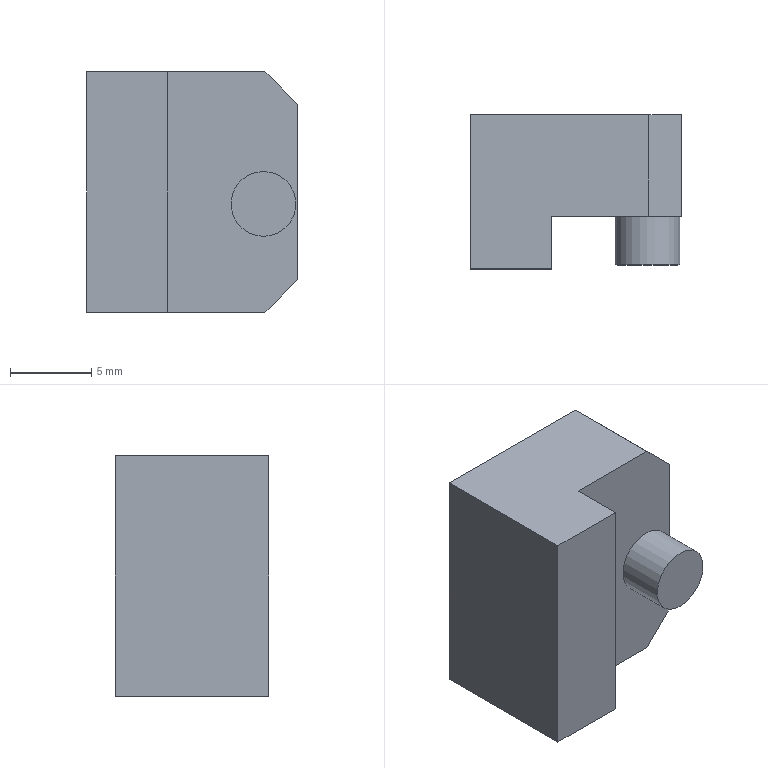Component | NX | SLIDER | 1 solid | 12 faces | box 13 x 9.5 x 14.83 mm | volume 1458 mm3 | plane 11 | cylinder 1 | commonest cylinder face diameters 4 x1
STEP:
#1=CARTESIAN_POINT('',(0.,0.,0.));
#2=DIRECTION('',(0.,0.,1.));
#3=DIRECTION('',(1.,0.,0.));
#4=AXIS2_PLACEMENT_3D('',#1,#2,#3);
#5=CARTESIAN_POINT('',(-316.,380.,341.346));
#6=VERTEX_POINT('',#5);
#7=CARTESIAN_POINT('',(-316.,380.,337.346));
#8=VERTEX_POINT('',#7);
#9=CARTESIAN_POINT('',(-316.,380.,339.346));
#10=DIRECTION('',(0.,-1.,0.));
#11=DIRECTION('',(0.,0.,1.));
#12=AXIS2_PLACEMENT_3D('',#9,#10,#11);
#13=CIRCLE('',#12,2.);
#14=CARTESIAN_POINT('',(-313.907,380.,347.493));
#15=DIRECTION('',(0.,1.,-0.));
#16=DIRECTION('',(0.,0.,1.));
#17=AXIS2_PLACEMENT_3D('',#14,#15,#16);
#18=PLANE('',#17);
#19=CARTESIAN_POINT('',(-6.147,-2.093));
#20=CARTESIAN_POINT('',(-6.147,-5.557));
#21=CARTESIAN_POINT('',(-9.147,-3.825));
#22=CARTESIAN_POINT('',(-12.147,-2.093));
#23=CARTESIAN_POINT('',(-9.147,-0.3606));
#24=CARTESIAN_POINT('',(-6.147,1.371));
#25=CARTESIAN_POINT('',(-6.147,-2.093));
#26=(BOUNDED_CURVE()B_SPLINE_CURVE(2,(#19,#20,#21,#22,#23,#24,#25),.UNSPECIFIED.,.T.,.F.)B_SPLINE_CURVE_WITH_KNOTS((1,2,2,2,2,1),(-2.094,0.,2.094,4.189,6.283,8.378),.UNSPECIFIED.)CURVE()GEOMETRIC_REPRESENTATION_ITEM()RATIONAL_B_SPLINE_CURVE((1.,0.5,1.,0.5,1.,0.5,1.))REPRESENTATION_ITEM(''));
#27=(GEOMETRIC_REPRESENTATION_CONTEXT(2)PARAMETRIC_REPRESENTATION_CONTEXT()REPRESENTATION_CONTEXT('',''));
#28=DEFINITIONAL_REPRESENTATION('',(#26),#27);
#29=PCURVE('',#18,#28);
#30=CARTESIAN_POINT('',(-316.,382.,339.346));
#31=DIRECTION('',(0.,-1.,-0.));
#32=DIRECTION('',(0.,0.,-1.));
#33=AXIS2_PLACEMENT_3D('',#30,#31,#32);
#34=CYLINDRICAL_SURFACE('',#33,2.);
#35=CARTESIAN_POINT('',(3.142,2.));
#36=DIRECTION('',(1.,0.));
#37=VECTOR('',#36,1.);
#38=LINE('',#35,#37);
#39=(GEOMETRIC_REPRESENTATION_CONTEXT(2)PARAMETRIC_REPRESENTATION_CONTEXT()REPRESENTATION_CONTEXT('',''));
#40=DEFINITIONAL_REPRESENTATION('',(#38),#39);
#41=PCURVE('',#34,#40);
#42=SURFACE_CURVE('',#13,(#29,#41),.PCURVE_S1.);
#43=EDGE_CURVE('',#6,#8,#42,.T.);
#44=ORIENTED_EDGE('',*,*,#43,.F.);
#45=CARTESIAN_POINT('',(-316.,380.,339.346));
#46=DIRECTION('',(0.,-1.,0.));
#47=DIRECTION('',(0.,0.,1.));
#48=AXIS2_PLACEMENT_3D('',#45,#46,#47);
#49=CIRCLE('',#48,2.);
#50=CARTESIAN_POINT('',(-6.147,-2.093));
#51=CARTESIAN_POINT('',(-6.147,-5.557));
#52=CARTESIAN_POINT('',(-9.147,-3.825));
#53=CARTESIAN_POINT('',(-12.147,-2.093));
#54=CARTESIAN_POINT('',(-9.147,-0.3606));
#55=CARTESIAN_POINT('',(-6.147,1.371));
#56=CARTESIAN_POINT('',(-6.147,-2.093));
#57=(BOUNDED_CURVE()B_SPLINE_CURVE(2,(#50,#51,#52,#53,#54,#55,#56),.UNSPECIFIED.,.T.,.F.)B_SPLINE_CURVE_WITH_KNOTS((1,2,2,2,2,1),(-2.094,0.,2.094,4.189,6.283,8.378),.UNSPECIFIED.)CURVE()GEOMETRIC_REPRESENTATION_ITEM()RATIONAL_B_SPLINE_CURVE((1.,0.5,1.,0.5,1.,0.5,1.))REPRESENTATION_ITEM(''));
#58=(GEOMETRIC_REPRESENTATION_CONTEXT(2)PARAMETRIC_REPRESENTATION_CONTEXT()REPRESENTATION_CONTEXT('',''));
#59=DEFINITIONAL_REPRESENTATION('',(#57),#58);
#60=PCURVE('',#18,#59);
#61=CARTESIAN_POINT('',(-3.142,2.));
#62=DIRECTION('',(1.,0.));
#63=VECTOR('',#62,1.);
#64=LINE('',#61,#63);
#65=(GEOMETRIC_REPRESENTATION_CONTEXT(2)PARAMETRIC_REPRESENTATION_CONTEXT()REPRESENTATION_CONTEXT('',''));
#66=DEFINITIONAL_REPRESENTATION('',(#64),#65);
#67=PCURVE('',#34,#66);
#68=SURFACE_CURVE('',#49,(#60,#67),.PCURVE_S1.);
#69=EDGE_CURVE('',#8,#6,#68,.T.);
#70=ORIENTED_EDGE('',*,*,#69,.F.);
#71=EDGE_LOOP('',(#44,#70));
#72=FACE_BOUND('',#71,.T.);
#73=CARTESIAN_POINT('',(-315.907,380.,332.665));
#74=VERTEX_POINT('',#73);
#75=CARTESIAN_POINT('',(-321.907,380.,332.665));
#76=VERTEX_POINT('',#75);
#77=CARTESIAN_POINT('',(-313.907,380.,332.665));
#78=DIRECTION('',(-1.,0.,0.));
#79=VECTOR('',#78,1.);
#80=LINE('',#77,#79);
#81=CARTESIAN_POINT('',(-14.828,0.));
#82=DIRECTION('',(0.,-1.));
#83=VECTOR('',#82,1.);
#84=LINE('',#81,#83);
#85=(GEOMETRIC_REPRESENTATION_CONTEXT(2)PARAMETRIC_REPRESENTATION_CONTEXT()REPRESENTATION_CONTEXT('',''));
#86=DEFINITIONAL_REPRESENTATION('',(#84),#85);
#87=PCURVE('',#18,#86);
#88=CARTESIAN_POINT('',(-313.907,380.,332.665));
#89=DIRECTION('',(0.,0.,1.));
#90=DIRECTION('',(-1.,0.,0.));
#91=AXIS2_PLACEMENT_3D('',#88,#89,#90);
#92=PLANE('',#91);
#93=CARTESIAN_POINT('',(0.,0.));
#94=DIRECTION('',(1.,0.));
#95=VECTOR('',#94,1.);
#96=LINE('',#93,#95);
#97=(GEOMETRIC_REPRESENTATION_CONTEXT(2)PARAMETRIC_REPRESENTATION_CONTEXT()REPRESENTATION_CONTEXT('',''));
#98=DEFINITIONAL_REPRESENTATION('',(#96),#97);
#99=PCURVE('',#92,#98);
#100=SURFACE_CURVE('',#80,(#87,#99),.PCURVE_S1.);
#101=EDGE_CURVE('',#74,#76,#100,.T.);
#102=ORIENTED_EDGE('',*,*,#101,.F.);
#103=CARTESIAN_POINT('',(-313.907,380.,334.665));
#104=VERTEX_POINT('',#103);
#105=CARTESIAN_POINT('',(-313.907,380.,334.665));
#106=DIRECTION('',(0.7071,0.,0.7071));
#107=VECTOR('',#106,1.);
#108=LINE('',#105,#107);
#109=CARTESIAN_POINT('',(-12.828,-0.));
#110=DIRECTION('',(0.7071,0.7071));
#111=VECTOR('',#110,1.);
#112=LINE('',#109,#111);
#113=(GEOMETRIC_REPRESENTATION_CONTEXT(2)PARAMETRIC_REPRESENTATION_CONTEXT()REPRESENTATION_CONTEXT('',''));
#114=DEFINITIONAL_REPRESENTATION('',(#112),#113);
#115=PCURVE('',#18,#114);
#116=CARTESIAN_POINT('',(-313.907,0.,334.665));
#117=DIRECTION('',(0.7071,0.,-0.7071));
#118=DIRECTION('',(0.,-1.,0.));
#119=AXIS2_PLACEMENT_3D('',#116,#117,#118);
#120=PLANE('',#119);
#121=CARTESIAN_POINT('',(-380.,0.));
#122=DIRECTION('',(-0.,-1.));
#123=VECTOR('',#122,1.);
#124=LINE('',#121,#123);
#125=(GEOMETRIC_REPRESENTATION_CONTEXT(2)PARAMETRIC_REPRESENTATION_CONTEXT()REPRESENTATION_CONTEXT('',''));
#126=DEFINITIONAL_REPRESENTATION('',(#124),#125);
#127=PCURVE('',#120,#126);
#128=SURFACE_CURVE('',#108,(#115,#127),.PCURVE_S1.);
#129=EDGE_CURVE('',#74,#104,#128,.T.);
#130=ORIENTED_EDGE('',*,*,#129,.T.);
#131=CARTESIAN_POINT('',(-313.907,380.,345.493));
#132=VERTEX_POINT('',#131);
#133=CARTESIAN_POINT('',(-313.907,380.,347.493));
#134=DIRECTION('',(0.,-0.,-1.));
#135=VECTOR('',#134,1.);
#136=LINE('',#133,#135);
#137=CARTESIAN_POINT('',(0.,0.));
#138=DIRECTION('',(-1.,0.));
#139=VECTOR('',#138,1.);
#140=LINE('',#137,#139);
#141=(GEOMETRIC_REPRESENTATION_CONTEXT(2)PARAMETRIC_REPRESENTATION_CONTEXT()REPRESENTATION_CONTEXT('',''));
#142=DEFINITIONAL_REPRESENTATION('',(#140),#141);
#143=PCURVE('',#18,#142);
#144=CARTESIAN_POINT('',(-313.907,0.,678.691));
#145=DIRECTION('',(1.,0.,0.));
#146=DIRECTION('',(0.,0.,1.));
#147=AXIS2_PLACEMENT_3D('',#144,#145,#146);
#148=PLANE('',#147);
#149=CARTESIAN_POINT('',(-331.198,-380.));
#150=DIRECTION('',(-1.,0.));
#151=VECTOR('',#150,1.);
#152=LINE('',#149,#151);
#153=(GEOMETRIC_REPRESENTATION_CONTEXT(2)PARAMETRIC_REPRESENTATION_CONTEXT()REPRESENTATION_CONTEXT('',''));
#154=DEFINITIONAL_REPRESENTATION('',(#152),#153);
#155=PCURVE('',#148,#154);
#156=SURFACE_CURVE('',#136,(#143,#155),.PCURVE_S1.);
#157=EDGE_CURVE('',#132,#104,#156,.T.);
#158=ORIENTED_EDGE('',*,*,#157,.F.);
#159=CARTESIAN_POINT('',(-315.907,380.,347.493));
#160=VERTEX_POINT('',#159);
#161=CARTESIAN_POINT('',(-313.907,380.,345.493));
#162=DIRECTION('',(-0.7071,0.,0.7071));
#163=VECTOR('',#162,1.);
#164=LINE('',#161,#163);
#165=CARTESIAN_POINT('',(-2.,0.));
#166=DIRECTION('',(0.7071,-0.7071));
#167=VECTOR('',#166,1.);
#168=LINE('',#165,#167);
#169=(GEOMETRIC_REPRESENTATION_CONTEXT(2)PARAMETRIC_REPRESENTATION_CONTEXT()REPRESENTATION_CONTEXT('',''));
#170=DEFINITIONAL_REPRESENTATION('',(#168),#169);
#171=PCURVE('',#18,#170);
#172=CARTESIAN_POINT('',(-313.907,0.,345.493));
#173=DIRECTION('',(0.7071,0.,0.7071));
#174=DIRECTION('',(0.,1.,0.));
#175=AXIS2_PLACEMENT_3D('',#172,#173,#174);
#176=PLANE('',#175);
#177=CARTESIAN_POINT('',(380.,-0.));
#178=DIRECTION('',(0.,1.));
#179=VECTOR('',#178,1.);
#180=LINE('',#177,#179);
#181=(GEOMETRIC_REPRESENTATION_CONTEXT(2)PARAMETRIC_REPRESENTATION_CONTEXT()REPRESENTATION_CONTEXT('',''));
#182=DEFINITIONAL_REPRESENTATION('',(#180),#181);
#183=PCURVE('',#176,#182);
#184=SURFACE_CURVE('',#164,(#171,#183),.PCURVE_S1.);
#185=EDGE_CURVE('',#132,#160,#184,.T.);
#186=ORIENTED_EDGE('',*,*,#185,.T.);
#187=CARTESIAN_POINT('',(-321.907,380.,347.493));
#188=VERTEX_POINT('',#187);
#189=CARTESIAN_POINT('',(-313.907,380.,347.493));
#190=DIRECTION('',(-1.,0.,0.));
#191=VECTOR('',#190,1.);
#192=LINE('',#189,#191);
#193=CARTESIAN_POINT('',(0.,0.));
#194=DIRECTION('',(0.,-1.));
#195=VECTOR('',#194,1.);
#196=LINE('',#193,#195);
#197=(GEOMETRIC_REPRESENTATION_CONTEXT(2)PARAMETRIC_REPRESENTATION_CONTEXT()REPRESENTATION_CONTEXT('',''));
#198=DEFINITIONAL_REPRESENTATION('',(#196),#197);
#199=PCURVE('',#18,#198);
#200=CARTESIAN_POINT('',(-313.907,386.248,347.493));
#201=DIRECTION('',(0.,0.,-1.));
#202=DIRECTION('',(1.,0.,0.));
#203=AXIS2_PLACEMENT_3D('',#200,#201,#202);
#204=PLANE('',#203);
#205=CARTESIAN_POINT('',(0.,6.248));
#206=DIRECTION('',(-1.,0.));
#207=VECTOR('',#206,1.);
#208=LINE('',#205,#207);
#209=(GEOMETRIC_REPRESENTATION_CONTEXT(2)PARAMETRIC_REPRESENTATION_CONTEXT()REPRESENTATION_CONTEXT('',''));
#210=DEFINITIONAL_REPRESENTATION('',(#208),#209);
#211=PCURVE('',#204,#210);
#212=SURFACE_CURVE('',#192,(#199,#211),.PCURVE_S1.);
#213=EDGE_CURVE('',#160,#188,#212,.T.);
#214=ORIENTED_EDGE('',*,*,#213,.T.);
#215=CARTESIAN_POINT('',(-321.907,380.,332.665));
#216=DIRECTION('',(0.,0.,1.));
#217=VECTOR('',#216,1.);
#218=LINE('',#215,#217);
#219=CARTESIAN_POINT('',(-14.828,-8.));
#220=DIRECTION('',(1.,0.));
#221=VECTOR('',#220,1.);
#222=LINE('',#219,#221);
#223=(GEOMETRIC_REPRESENTATION_CONTEXT(2)PARAMETRIC_REPRESENTATION_CONTEXT()REPRESENTATION_CONTEXT('',''));
#224=DEFINITIONAL_REPRESENTATION('',(#222),#223);
#225=PCURVE('',#18,#224);
#226=CARTESIAN_POINT('',(-321.907,0.,678.691));
#227=DIRECTION('',(1.,0.,0.));
#228=DIRECTION('',(0.,0.,1.));
#229=AXIS2_PLACEMENT_3D('',#226,#227,#228);
#230=PLANE('',#229);
#231=CARTESIAN_POINT('',(-346.026,-380.));
#232=DIRECTION('',(1.,-0.));
#233=VECTOR('',#232,1.);
#234=LINE('',#231,#233);
#235=(GEOMETRIC_REPRESENTATION_CONTEXT(2)PARAMETRIC_REPRESENTATION_CONTEXT()REPRESENTATION_CONTEXT('',''));
#236=DEFINITIONAL_REPRESENTATION('',(#234),#235);
#237=PCURVE('',#230,#236);
#238=SURFACE_CURVE('',#218,(#225,#237),.PCURVE_S1.);
#239=EDGE_CURVE('',#76,#188,#238,.T.);
#240=ORIENTED_EDGE('',*,*,#239,.F.);
#241=EDGE_LOOP('',(#102,#130,#158,#186,#214,#240));
#242=FACE_BOUND('',#241,.T.);
#243=ADVANCED_FACE('',(#72,#242),#18,.F.);
#244=CARTESIAN_POINT('',(-313.907,386.248,334.665));
#245=VERTEX_POINT('',#244);
#246=CARTESIAN_POINT('',(-313.907,386.248,345.493));
#247=VERTEX_POINT('',#246);
#248=CARTESIAN_POINT('',(-313.907,386.248,332.665));
#249=DIRECTION('',(0.,0.,1.));
#250=VECTOR('',#249,1.);
#251=LINE('',#248,#250);
#252=CARTESIAN_POINT('',(-313.907,386.248,332.665));
#253=DIRECTION('',(0.,-1.,0.));
#254=DIRECTION('',(0.,0.,-1.));
#255=AXIS2_PLACEMENT_3D('',#252,#253,#254);
#256=PLANE('',#255);
#257=CARTESIAN_POINT('',(0.,0.));
#258=DIRECTION('',(-1.,0.));
#259=VECTOR('',#258,1.);
#260=LINE('',#257,#259);
#261=(GEOMETRIC_REPRESENTATION_CONTEXT(2)PARAMETRIC_REPRESENTATION_CONTEXT()REPRESENTATION_CONTEXT('',''));
#262=DEFINITIONAL_REPRESENTATION('',(#260),#261);
#263=PCURVE('',#256,#262);
#264=CARTESIAN_POINT('',(-346.026,-386.248));
#265=DIRECTION('',(1.,0.));
#266=VECTOR('',#265,1.);
#267=LINE('',#264,#266);
#268=(GEOMETRIC_REPRESENTATION_CONTEXT(2)PARAMETRIC_REPRESENTATION_CONTEXT()REPRESENTATION_CONTEXT('',''));
#269=DEFINITIONAL_REPRESENTATION('',(#267),#268);
#270=PCURVE('',#148,#269);
#271=SURFACE_CURVE('',#251,(#263,#270),.PCURVE_S1.);
#272=EDGE_CURVE('',#245,#247,#271,.T.);
#273=ORIENTED_EDGE('',*,*,#272,.F.);
#274=CARTESIAN_POINT('',(-315.907,386.248,332.665));
#275=VERTEX_POINT('',#274);
#276=CARTESIAN_POINT('',(-313.907,386.248,334.665));
#277=DIRECTION('',(-0.7071,0.,-0.7071));
#278=VECTOR('',#277,1.);
#279=LINE('',#276,#278);
#280=CARTESIAN_POINT('',(-2.,0.));
#281=DIRECTION('',(0.7071,-0.7071));
#282=VECTOR('',#281,1.);
#283=LINE('',#280,#282);
#284=(GEOMETRIC_REPRESENTATION_CONTEXT(2)PARAMETRIC_REPRESENTATION_CONTEXT()REPRESENTATION_CONTEXT('',''));
#285=DEFINITIONAL_REPRESENTATION('',(#283),#284);
#286=PCURVE('',#256,#285);
#287=CARTESIAN_POINT('',(-386.248,0.));
#288=DIRECTION('',(0.,1.));
#289=VECTOR('',#288,1.);
#290=LINE('',#287,#289);
#291=(GEOMETRIC_REPRESENTATION_CONTEXT(2)PARAMETRIC_REPRESENTATION_CONTEXT()REPRESENTATION_CONTEXT('',''));
#292=DEFINITIONAL_REPRESENTATION('',(#290),#291);
#293=PCURVE('',#120,#292);
#294=SURFACE_CURVE('',#279,(#286,#293),.PCURVE_S1.);
#295=EDGE_CURVE('',#245,#275,#294,.T.);
#296=ORIENTED_EDGE('',*,*,#295,.T.);
#297=CARTESIAN_POINT('',(-326.907,386.248,332.665));
#298=VERTEX_POINT('',#297);
#299=CARTESIAN_POINT('',(-313.907,386.248,332.665));
#300=DIRECTION('',(-1.,0.,0.));
#301=VECTOR('',#300,1.);
#302=LINE('',#299,#301);
#303=CARTESIAN_POINT('',(0.,0.));
#304=DIRECTION('',(0.,-1.));
#305=VECTOR('',#304,1.);
#306=LINE('',#303,#305);
#307=(GEOMETRIC_REPRESENTATION_CONTEXT(2)PARAMETRIC_REPRESENTATION_CONTEXT()REPRESENTATION_CONTEXT('',''));
#308=DEFINITIONAL_REPRESENTATION('',(#306),#307);
#309=PCURVE('',#256,#308);
#310=CARTESIAN_POINT('',(0.,-6.248));
#311=DIRECTION('',(1.,0.));
#312=VECTOR('',#311,1.);
#313=LINE('',#310,#312);
#314=(GEOMETRIC_REPRESENTATION_CONTEXT(2)PARAMETRIC_REPRESENTATION_CONTEXT()REPRESENTATION_CONTEXT('',''));
#315=DEFINITIONAL_REPRESENTATION('',(#313),#314);
#316=PCURVE('',#92,#315);
#317=SURFACE_CURVE('',#302,(#309,#316),.PCURVE_S1.);
#318=EDGE_CURVE('',#275,#298,#317,.T.);
#319=ORIENTED_EDGE('',*,*,#318,.T.);
#320=CARTESIAN_POINT('',(-326.907,386.248,347.493));
#321=VERTEX_POINT('',#320);
#322=CARTESIAN_POINT('',(-326.907,386.248,332.665));
#323=DIRECTION('',(0.,0.,1.));
#324=VECTOR('',#323,1.);
#325=LINE('',#322,#324);
#326=CARTESIAN_POINT('',(0.,-13.));
#327=DIRECTION('',(-1.,0.));
#328=VECTOR('',#327,1.);
#329=LINE('',#326,#328);
#330=(GEOMETRIC_REPRESENTATION_CONTEXT(2)PARAMETRIC_REPRESENTATION_CONTEXT()REPRESENTATION_CONTEXT('',''));
#331=DEFINITIONAL_REPRESENTATION('',(#329),#330);
#332=PCURVE('',#256,#331);
#333=CARTESIAN_POINT('',(-326.907,386.248,8.691));
#334=DIRECTION('',(-1.,0.,0.));
#335=DIRECTION('',(0.,0.,-1.));
#336=AXIS2_PLACEMENT_3D('',#333,#334,#335);
#337=PLANE('',#336);
#338=CARTESIAN_POINT('',(-323.974,0.));
#339=DIRECTION('',(-1.,0.));
#340=VECTOR('',#339,1.);
#341=LINE('',#338,#340);
#342=(GEOMETRIC_REPRESENTATION_CONTEXT(2)PARAMETRIC_REPRESENTATION_CONTEXT()REPRESENTATION_CONTEXT('',''));
#343=DEFINITIONAL_REPRESENTATION('',(#341),#342);
#344=PCURVE('',#337,#343);
#345=SURFACE_CURVE('',#325,(#332,#344),.PCURVE_S1.);
#346=EDGE_CURVE('',#298,#321,#345,.T.);
#347=ORIENTED_EDGE('',*,*,#346,.T.);
#348=CARTESIAN_POINT('',(-315.907,386.248,347.493));
#349=VERTEX_POINT('',#348);
#350=CARTESIAN_POINT('',(-313.907,386.248,347.493));
#351=DIRECTION('',(-1.,0.,0.));
#352=VECTOR('',#351,1.);
#353=LINE('',#350,#352);
#354=CARTESIAN_POINT('',(-14.828,0.));
#355=DIRECTION('',(0.,-1.));
#356=VECTOR('',#355,1.);
#357=LINE('',#354,#356);
#358=(GEOMETRIC_REPRESENTATION_CONTEXT(2)PARAMETRIC_REPRESENTATION_CONTEXT()REPRESENTATION_CONTEXT('',''));
#359=DEFINITIONAL_REPRESENTATION('',(#357),#358);
#360=PCURVE('',#256,#359);
#361=CARTESIAN_POINT('',(0.,0.));
#362=DIRECTION('',(-1.,0.));
#363=VECTOR('',#362,1.);
#364=LINE('',#361,#363);
#365=(GEOMETRIC_REPRESENTATION_CONTEXT(2)PARAMETRIC_REPRESENTATION_CONTEXT()REPRESENTATION_CONTEXT('',''));
#366=DEFINITIONAL_REPRESENTATION('',(#364),#365);
#367=PCURVE('',#204,#366);
#368=SURFACE_CURVE('',#353,(#360,#367),.PCURVE_S1.);
#369=EDGE_CURVE('',#349,#321,#368,.T.);
#370=ORIENTED_EDGE('',*,*,#369,.F.);
#371=CARTESIAN_POINT('',(-313.907,386.248,345.493));
#372=DIRECTION('',(0.7071,0.,-0.7071));
#373=VECTOR('',#372,1.);
#374=LINE('',#371,#373);
#375=CARTESIAN_POINT('',(-12.828,0.));
#376=DIRECTION('',(0.7071,0.7071));
#377=VECTOR('',#376,1.);
#378=LINE('',#375,#377);
#379=(GEOMETRIC_REPRESENTATION_CONTEXT(2)PARAMETRIC_REPRESENTATION_CONTEXT()REPRESENTATION_CONTEXT('',''));
#380=DEFINITIONAL_REPRESENTATION('',(#378),#379);
#381=PCURVE('',#256,#380);
#382=CARTESIAN_POINT('',(386.248,0.));
#383=DIRECTION('',(0.,-1.));
#384=VECTOR('',#383,1.);
#385=LINE('',#382,#384);
#386=(GEOMETRIC_REPRESENTATION_CONTEXT(2)PARAMETRIC_REPRESENTATION_CONTEXT()REPRESENTATION_CONTEXT('',''));
#387=DEFINITIONAL_REPRESENTATION('',(#385),#386);
#388=PCURVE('',#176,#387);
#389=SURFACE_CURVE('',#374,(#381,#388),.PCURVE_S1.);
#390=EDGE_CURVE('',#349,#247,#389,.T.);
#391=ORIENTED_EDGE('',*,*,#390,.T.);
#392=EDGE_LOOP('',(#273,#296,#319,#347,#370,#391));
#393=FACE_BOUND('',#392,.T.);
#394=ADVANCED_FACE('',(#393),#256,.F.);
#395=ORIENTED_EDGE('',*,*,#213,.F.);
#396=CARTESIAN_POINT('',(-315.907,386.248,347.493));
#397=DIRECTION('',(0.,1.,0.));
#398=VECTOR('',#397,1.);
#399=LINE('',#396,#398);
#400=CARTESIAN_POINT('',(-2.,0.));
#401=DIRECTION('',(0.,-1.));
#402=VECTOR('',#401,1.);
#403=LINE('',#400,#402);
#404=(GEOMETRIC_REPRESENTATION_CONTEXT(2)PARAMETRIC_REPRESENTATION_CONTEXT()REPRESENTATION_CONTEXT('',''));
#405=DEFINITIONAL_REPRESENTATION('',(#403),#404);
#406=PCURVE('',#204,#405);
#407=CARTESIAN_POINT('',(386.248,2.828));
#408=DIRECTION('',(1.,0.));
#409=VECTOR('',#408,1.);
#410=LINE('',#407,#409);
#411=(GEOMETRIC_REPRESENTATION_CONTEXT(2)PARAMETRIC_REPRESENTATION_CONTEXT()REPRESENTATION_CONTEXT('',''));
#412=DEFINITIONAL_REPRESENTATION('',(#410),#411);
#413=PCURVE('',#176,#412);
#414=SURFACE_CURVE('',#399,(#406,#413),.PCURVE_S1.);
#415=EDGE_CURVE('',#160,#349,#414,.T.);
#416=ORIENTED_EDGE('',*,*,#415,.T.);
#417=ORIENTED_EDGE('',*,*,#369,.T.);
#418=CARTESIAN_POINT('',(-326.907,376.752,347.493));
#419=VERTEX_POINT('',#418);
#420=CARTESIAN_POINT('',(-326.907,386.248,347.493));
#421=DIRECTION('',(0.,-1.,0.));
#422=VECTOR('',#421,1.);
#423=LINE('',#420,#422);
#424=CARTESIAN_POINT('',(-13.,0.));
#425=DIRECTION('',(0.,1.));
#426=VECTOR('',#425,1.);
#427=LINE('',#424,#426);
#428=(GEOMETRIC_REPRESENTATION_CONTEXT(2)PARAMETRIC_REPRESENTATION_CONTEXT()REPRESENTATION_CONTEXT('',''));
#429=DEFINITIONAL_REPRESENTATION('',(#427),#428);
#430=PCURVE('',#204,#429);
#431=CARTESIAN_POINT('',(-338.802,0.));
#432=DIRECTION('',(0.,1.));
#433=VECTOR('',#432,1.);
#434=LINE('',#431,#433);
#435=(GEOMETRIC_REPRESENTATION_CONTEXT(2)PARAMETRIC_REPRESENTATION_CONTEXT()REPRESENTATION_CONTEXT('',''));
#436=DEFINITIONAL_REPRESENTATION('',(#434),#435);
#437=PCURVE('',#337,#436);
#438=SURFACE_CURVE('',#423,(#430,#437),.PCURVE_S1.);
#439=EDGE_CURVE('',#321,#419,#438,.T.);
#440=ORIENTED_EDGE('',*,*,#439,.T.);
#441=CARTESIAN_POINT('',(-321.907,376.752,347.493));
#442=VERTEX_POINT('',#441);
#443=CARTESIAN_POINT('',(-326.907,376.752,347.493));
#444=DIRECTION('',(1.,0.,0.));
#445=VECTOR('',#444,1.);
#446=LINE('',#443,#445);
#447=CARTESIAN_POINT('',(-13.,9.496));
#448=DIRECTION('',(1.,0.));
#449=VECTOR('',#448,1.);
#450=LINE('',#447,#449);
#451=(GEOMETRIC_REPRESENTATION_CONTEXT(2)PARAMETRIC_REPRESENTATION_CONTEXT()REPRESENTATION_CONTEXT('',''));
#452=DEFINITIONAL_REPRESENTATION('',(#450),#451);
#453=PCURVE('',#204,#452);
#454=CARTESIAN_POINT('',(-326.907,376.752,347.493));
#455=DIRECTION('',(0.,-1.,0.));
#456=DIRECTION('',(0.,0.,-1.));
#457=AXIS2_PLACEMENT_3D('',#454,#455,#456);
#458=PLANE('',#457);
#459=CARTESIAN_POINT('',(0.,0.));
#460=DIRECTION('',(0.,1.));
#461=VECTOR('',#460,1.);
#462=LINE('',#459,#461);
#463=(GEOMETRIC_REPRESENTATION_CONTEXT(2)PARAMETRIC_REPRESENTATION_CONTEXT()REPRESENTATION_CONTEXT('',''));
#464=DEFINITIONAL_REPRESENTATION('',(#462),#463);
#465=PCURVE('',#458,#464);
#466=SURFACE_CURVE('',#446,(#453,#465),.PCURVE_S1.);
#467=EDGE_CURVE('',#419,#442,#466,.T.);
#468=ORIENTED_EDGE('',*,*,#467,.T.);
#469=CARTESIAN_POINT('',(-321.907,380.,347.493));
#470=DIRECTION('',(0.,-1.,0.));
#471=VECTOR('',#470,1.);
#472=LINE('',#469,#471);
#473=CARTESIAN_POINT('',(-8.,6.248));
#474=DIRECTION('',(0.,1.));
#475=VECTOR('',#474,1.);
#476=LINE('',#473,#475);
#477=(GEOMETRIC_REPRESENTATION_CONTEXT(2)PARAMETRIC_REPRESENTATION_CONTEXT()REPRESENTATION_CONTEXT('',''));
#478=DEFINITIONAL_REPRESENTATION('',(#476),#477);
#479=PCURVE('',#204,#478);
#480=CARTESIAN_POINT('',(-331.198,-380.));
#481=DIRECTION('',(0.,1.));
#482=VECTOR('',#481,1.);
#483=LINE('',#480,#482);
#484=(GEOMETRIC_REPRESENTATION_CONTEXT(2)PARAMETRIC_REPRESENTATION_CONTEXT()REPRESENTATION_CONTEXT('',''));
#485=DEFINITIONAL_REPRESENTATION('',(#483),#484);
#486=PCURVE('',#230,#485);
#487=SURFACE_CURVE('',#472,(#479,#486),.PCURVE_S1.);
#488=EDGE_CURVE('',#188,#442,#487,.T.);
#489=ORIENTED_EDGE('',*,*,#488,.F.);
#490=EDGE_LOOP('',(#395,#416,#417,#440,#468,#489));
#491=FACE_BOUND('',#490,.T.);
#492=ADVANCED_FACE('',(#491),#204,.F.);
#493=ORIENTED_EDGE('',*,*,#318,.F.);
#494=CARTESIAN_POINT('',(-315.907,380.,332.665));
#495=DIRECTION('',(0.,-1.,0.));
#496=VECTOR('',#495,1.);
#497=LINE('',#494,#496);
#498=CARTESIAN_POINT('',(2.,0.));
#499=DIRECTION('',(0.,1.));
#500=VECTOR('',#499,1.);
#501=LINE('',#498,#500);
#502=(GEOMETRIC_REPRESENTATION_CONTEXT(2)PARAMETRIC_REPRESENTATION_CONTEXT()REPRESENTATION_CONTEXT('',''));
#503=DEFINITIONAL_REPRESENTATION('',(#501),#502);
#504=PCURVE('',#92,#503);
#505=CARTESIAN_POINT('',(-380.,2.828));
#506=DIRECTION('',(1.,0.));
#507=VECTOR('',#506,1.);
#508=LINE('',#505,#507);
#509=(GEOMETRIC_REPRESENTATION_CONTEXT(2)PARAMETRIC_REPRESENTATION_CONTEXT()REPRESENTATION_CONTEXT('',''));
#510=DEFINITIONAL_REPRESENTATION('',(#508),#509);
#511=PCURVE('',#120,#510);
#512=SURFACE_CURVE('',#497,(#504,#511),.PCURVE_S1.);
#513=EDGE_CURVE('',#275,#74,#512,.T.);
#514=ORIENTED_EDGE('',*,*,#513,.T.);
#515=ORIENTED_EDGE('',*,*,#101,.T.);
#516=CARTESIAN_POINT('',(-321.907,376.752,332.665));
#517=VERTEX_POINT('',#516);
#518=CARTESIAN_POINT('',(-321.907,376.752,332.665));
#519=DIRECTION('',(0.,1.,0.));
#520=VECTOR('',#519,1.);
#521=LINE('',#518,#520);
#522=CARTESIAN_POINT('',(8.,3.248));
#523=DIRECTION('',(0.,-1.));
#524=VECTOR('',#523,1.);
#525=LINE('',#522,#524);
#526=(GEOMETRIC_REPRESENTATION_CONTEXT(2)PARAMETRIC_REPRESENTATION_CONTEXT()REPRESENTATION_CONTEXT('',''));
#527=DEFINITIONAL_REPRESENTATION('',(#525),#526);
#528=PCURVE('',#92,#527);
#529=CARTESIAN_POINT('',(-346.026,-376.752));
#530=DIRECTION('',(0.,-1.));
#531=VECTOR('',#530,1.);
#532=LINE('',#529,#531);
#533=(GEOMETRIC_REPRESENTATION_CONTEXT(2)PARAMETRIC_REPRESENTATION_CONTEXT()REPRESENTATION_CONTEXT('',''));
#534=DEFINITIONAL_REPRESENTATION('',(#532),#533);
#535=PCURVE('',#230,#534);
#536=SURFACE_CURVE('',#521,(#528,#535),.PCURVE_S1.);
#537=EDGE_CURVE('',#517,#76,#536,.T.);
#538=ORIENTED_EDGE('',*,*,#537,.F.);
#539=CARTESIAN_POINT('',(-326.907,376.752,332.665));
#540=VERTEX_POINT('',#539);
#541=CARTESIAN_POINT('',(-326.907,376.752,332.665));
#542=DIRECTION('',(1.,0.,0.));
#543=VECTOR('',#542,1.);
#544=LINE('',#541,#543);
#545=CARTESIAN_POINT('',(13.,3.248));
#546=DIRECTION('',(-1.,0.));
#547=VECTOR('',#546,1.);
#548=LINE('',#545,#547);
#549=(GEOMETRIC_REPRESENTATION_CONTEXT(2)PARAMETRIC_REPRESENTATION_CONTEXT()REPRESENTATION_CONTEXT('',''));
#550=DEFINITIONAL_REPRESENTATION('',(#548),#549);
#551=PCURVE('',#92,#550);
#552=CARTESIAN_POINT('',(14.828,0.));
#553=DIRECTION('',(0.,1.));
#554=VECTOR('',#553,1.);
#555=LINE('',#552,#554);
#556=(GEOMETRIC_REPRESENTATION_CONTEXT(2)PARAMETRIC_REPRESENTATION_CONTEXT()REPRESENTATION_CONTEXT('',''));
#557=DEFINITIONAL_REPRESENTATION('',(#555),#556);
#558=PCURVE('',#458,#557);
#559=SURFACE_CURVE('',#544,(#551,#558),.PCURVE_S1.);
#560=EDGE_CURVE('',#540,#517,#559,.T.);
#561=ORIENTED_EDGE('',*,*,#560,.F.);
#562=CARTESIAN_POINT('',(-326.907,380.,332.665));
#563=DIRECTION('',(0.,1.,0.));
#564=VECTOR('',#563,1.);
#565=LINE('',#562,#564);
#566=CARTESIAN_POINT('',(13.,0.));
#567=DIRECTION('',(0.,-1.));
#568=VECTOR('',#567,1.);
#569=LINE('',#566,#568);
#570=(GEOMETRIC_REPRESENTATION_CONTEXT(2)PARAMETRIC_REPRESENTATION_CONTEXT()REPRESENTATION_CONTEXT('',''));
#571=DEFINITIONAL_REPRESENTATION('',(#569),#570);
#572=PCURVE('',#92,#571);
#573=CARTESIAN_POINT('',(-323.974,6.248));
#574=DIRECTION('',(0.,-1.));
#575=VECTOR('',#574,1.);
#576=LINE('',#573,#575);
#577=(GEOMETRIC_REPRESENTATION_CONTEXT(2)PARAMETRIC_REPRESENTATION_CONTEXT()REPRESENTATION_CONTEXT('',''));
#578=DEFINITIONAL_REPRESENTATION('',(#576),#577);
#579=PCURVE('',#337,#578);
#580=SURFACE_CURVE('',#565,(#572,#579),.PCURVE_S1.);
#581=EDGE_CURVE('',#540,#298,#580,.T.);
#582=ORIENTED_EDGE('',*,*,#581,.T.);
#583=EDGE_LOOP('',(#493,#514,#515,#538,#561,#582));
#584=FACE_BOUND('',#583,.T.);
#585=ADVANCED_FACE('',(#584),#92,.F.);
#586=ORIENTED_EDGE('',*,*,#157,.T.);
#587=CARTESIAN_POINT('',(-313.907,386.248,334.665));
#588=DIRECTION('',(0.,1.,0.));
#589=VECTOR('',#588,1.);
#590=LINE('',#587,#589);
#591=CARTESIAN_POINT('',(-344.026,-386.248));
#592=DIRECTION('',(0.,-1.));
#593=VECTOR('',#592,1.);
#594=LINE('',#591,#593);
#595=(GEOMETRIC_REPRESENTATION_CONTEXT(2)PARAMETRIC_REPRESENTATION_CONTEXT()REPRESENTATION_CONTEXT('',''));
#596=DEFINITIONAL_REPRESENTATION('',(#594),#595);
#597=PCURVE('',#148,#596);
#598=CARTESIAN_POINT('',(-386.248,0.));
#599=DIRECTION('',(-1.,0.));
#600=VECTOR('',#599,1.);
#601=LINE('',#598,#600);
#602=(GEOMETRIC_REPRESENTATION_CONTEXT(2)PARAMETRIC_REPRESENTATION_CONTEXT()REPRESENTATION_CONTEXT('',''));
#603=DEFINITIONAL_REPRESENTATION('',(#601),#602);
#604=PCURVE('',#120,#603);
#605=SURFACE_CURVE('',#590,(#597,#604),.PCURVE_S1.);
#606=EDGE_CURVE('',#104,#245,#605,.T.);
#607=ORIENTED_EDGE('',*,*,#606,.T.);
#608=ORIENTED_EDGE('',*,*,#272,.T.);
#609=CARTESIAN_POINT('',(-313.907,380.,345.493));
#610=DIRECTION('',(0.,-1.,0.));
#611=VECTOR('',#610,1.);
#612=LINE('',#609,#611);
#613=CARTESIAN_POINT('',(-333.198,-380.));
#614=DIRECTION('',(0.,1.));
#615=VECTOR('',#614,1.);
#616=LINE('',#613,#615);
#617=(GEOMETRIC_REPRESENTATION_CONTEXT(2)PARAMETRIC_REPRESENTATION_CONTEXT()REPRESENTATION_CONTEXT('',''));
#618=DEFINITIONAL_REPRESENTATION('',(#616),#617);
#619=PCURVE('',#148,#618);
#620=CARTESIAN_POINT('',(380.,0.));
#621=DIRECTION('',(-1.,0.));
#622=VECTOR('',#621,1.);
#623=LINE('',#620,#622);
#624=(GEOMETRIC_REPRESENTATION_CONTEXT(2)PARAMETRIC_REPRESENTATION_CONTEXT()REPRESENTATION_CONTEXT('',''));
#625=DEFINITIONAL_REPRESENTATION('',(#623),#624);
#626=PCURVE('',#176,#625);
#627=SURFACE_CURVE('',#612,(#619,#626),.PCURVE_S1.);
#628=EDGE_CURVE('',#247,#132,#627,.T.);
#629=ORIENTED_EDGE('',*,*,#628,.T.);
#630=EDGE_LOOP('',(#586,#607,#608,#629));
#631=FACE_BOUND('',#630,.T.);
#632=ADVANCED_FACE('',(#631),#148,.T.);
#633=ORIENTED_EDGE('',*,*,#346,.F.);
#634=ORIENTED_EDGE('',*,*,#581,.F.);
#635=CARTESIAN_POINT('',(-326.907,376.752,347.493));
#636=DIRECTION('',(0.,0.,-1.));
#637=VECTOR('',#636,1.);
#638=LINE('',#635,#637);
#639=CARTESIAN_POINT('',(-338.802,9.496));
#640=DIRECTION('',(1.,0.));
#641=VECTOR('',#640,1.);
#642=LINE('',#639,#641);
#643=(GEOMETRIC_REPRESENTATION_CONTEXT(2)PARAMETRIC_REPRESENTATION_CONTEXT()REPRESENTATION_CONTEXT('',''));
#644=DEFINITIONAL_REPRESENTATION('',(#642),#643);
#645=PCURVE('',#337,#644);
#646=CARTESIAN_POINT('',(0.,0.));
#647=DIRECTION('',(1.,0.));
#648=VECTOR('',#647,1.);
#649=LINE('',#646,#648);
#650=(GEOMETRIC_REPRESENTATION_CONTEXT(2)PARAMETRIC_REPRESENTATION_CONTEXT()REPRESENTATION_CONTEXT('',''));
#651=DEFINITIONAL_REPRESENTATION('',(#649),#650);
#652=PCURVE('',#458,#651);
#653=SURFACE_CURVE('',#638,(#645,#652),.PCURVE_S1.);
#654=EDGE_CURVE('',#419,#540,#653,.T.);
#655=ORIENTED_EDGE('',*,*,#654,.F.);
#656=ORIENTED_EDGE('',*,*,#439,.F.);
#657=EDGE_LOOP('',(#633,#634,#655,#656));
#658=FACE_BOUND('',#657,.T.);
#659=ADVANCED_FACE('',(#658),#337,.T.);
#660=CARTESIAN_POINT('',(-321.907,376.752,347.493));
#661=DIRECTION('',(0.,0.,-1.));
#662=VECTOR('',#661,1.);
#663=LINE('',#660,#662);
#664=CARTESIAN_POINT('',(0.,5.));
#665=DIRECTION('',(1.,0.));
#666=VECTOR('',#665,1.);
#667=LINE('',#664,#666);
#668=(GEOMETRIC_REPRESENTATION_CONTEXT(2)PARAMETRIC_REPRESENTATION_CONTEXT()REPRESENTATION_CONTEXT('',''));
#669=DEFINITIONAL_REPRESENTATION('',(#667),#668);
#670=PCURVE('',#458,#669);
#671=CARTESIAN_POINT('',(-331.198,-376.752));
#672=DIRECTION('',(-1.,0.));
#673=VECTOR('',#672,1.);
#674=LINE('',#671,#673);
#675=(GEOMETRIC_REPRESENTATION_CONTEXT(2)PARAMETRIC_REPRESENTATION_CONTEXT()REPRESENTATION_CONTEXT('',''));
#676=DEFINITIONAL_REPRESENTATION('',(#674),#675);
#677=PCURVE('',#230,#676);
#678=SURFACE_CURVE('',#663,(#670,#677),.PCURVE_S1.);
#679=EDGE_CURVE('',#442,#517,#678,.T.);
#680=ORIENTED_EDGE('',*,*,#679,.F.);
#681=ORIENTED_EDGE('',*,*,#467,.F.);
#682=ORIENTED_EDGE('',*,*,#654,.T.);
#683=ORIENTED_EDGE('',*,*,#560,.T.);
#684=EDGE_LOOP('',(#680,#681,#682,#683));
#685=FACE_BOUND('',#684,.T.);
#686=ADVANCED_FACE('',(#685),#458,.T.);
#687=ORIENTED_EDGE('',*,*,#239,.T.);
#688=ORIENTED_EDGE('',*,*,#488,.T.);
#689=ORIENTED_EDGE('',*,*,#679,.T.);
#690=ORIENTED_EDGE('',*,*,#537,.T.);
#691=EDGE_LOOP('',(#687,#688,#689,#690));
#692=FACE_BOUND('',#691,.T.);
#693=ADVANCED_FACE('',(#692),#230,.T.);
#694=CARTESIAN_POINT('',(-316.,377.,337.346));
#695=VERTEX_POINT('',#694);
#696=CARTESIAN_POINT('',(-316.,377.,339.346));
#697=DIRECTION('',(0.,1.,0.));
#698=DIRECTION('',(0.,0.,-1.));
#699=AXIS2_PLACEMENT_3D('',#696,#697,#698);
#700=CIRCLE('',#699,2.);
#701=CARTESIAN_POINT('',(6.283,5.));
#702=DIRECTION('',(-1.,0.));
#703=VECTOR('',#702,1.);
#704=LINE('',#701,#703);
#705=(GEOMETRIC_REPRESENTATION_CONTEXT(2)PARAMETRIC_REPRESENTATION_CONTEXT()REPRESENTATION_CONTEXT('',''));
#706=DEFINITIONAL_REPRESENTATION('',(#704),#705);
#707=PCURVE('',#34,#706);
#708=CARTESIAN_POINT('',(-316.,377.,339.346));
#709=DIRECTION('',(0.,1.,0.));
#710=DIRECTION('',(0.,-0.,1.));
#711=AXIS2_PLACEMENT_3D('',#708,#709,#710);
#712=PLANE('',#711);
#713=CARTESIAN_POINT('',(0.,0.));
#714=DIRECTION('',(-1.,0.));
#715=AXIS2_PLACEMENT_2D('',#713,#714);
#716=CIRCLE('',#715,2.);
#717=(GEOMETRIC_REPRESENTATION_CONTEXT(2)PARAMETRIC_REPRESENTATION_CONTEXT()REPRESENTATION_CONTEXT('',''));
#718=DEFINITIONAL_REPRESENTATION('',(#716),#717);
#719=PCURVE('',#712,#718);
#720=SURFACE_CURVE('',#700,(#707,#719),.PCURVE_S1.);
#721=EDGE_CURVE('',#695,#695,#720,.T.);
#722=ORIENTED_EDGE('',*,*,#721,.T.);
#723=CARTESIAN_POINT('',(-316.,380.,337.346));
#724=CARTESIAN_POINT('',(-316.,377.,337.346));
#725=B_SPLINE_CURVE_WITH_KNOTS('',1,(#723,#724),.UNSPECIFIED.,.F.,.F.,(2,2),(2.,5.),.PIECEWISE_BEZIER_KNOTS.);
#726=CARTESIAN_POINT('',(0.,0.));
#727=DIRECTION('',(0.,1.));
#728=VECTOR('',#727,1.);
#729=LINE('',#726,#728);
#730=(GEOMETRIC_REPRESENTATION_CONTEXT(2)PARAMETRIC_REPRESENTATION_CONTEXT()REPRESENTATION_CONTEXT('',''));
#731=DEFINITIONAL_REPRESENTATION('',(#729),#730);
#732=PCURVE('',#34,#731);
#733=CARTESIAN_POINT('',(6.283,0.));
#734=DIRECTION('',(0.,1.));
#735=VECTOR('',#734,1.);
#736=LINE('',#733,#735);
#737=(GEOMETRIC_REPRESENTATION_CONTEXT(2)PARAMETRIC_REPRESENTATION_CONTEXT()REPRESENTATION_CONTEXT('',''));
#738=DEFINITIONAL_REPRESENTATION('',(#736),#737);
#739=PCURVE('',#34,#738);
#740=SEAM_CURVE('',#725,(#732,#739),.PCURVE_S1.);
#741=EDGE_CURVE('',#8,#695,#740,.T.);
#742=ORIENTED_EDGE('',*,*,#741,.F.);
#743=ORIENTED_EDGE('',*,*,#69,.T.);
#744=ORIENTED_EDGE('',*,*,#43,.T.);
#745=ORIENTED_EDGE('',*,*,#741,.T.);
#746=EDGE_LOOP('',(#722,#742,#743,#744,#745));
#747=FACE_BOUND('',#746,.T.);
#748=ADVANCED_FACE('',(#747),#34,.T.);
#749=ORIENTED_EDGE('',*,*,#721,.F.);
#750=EDGE_LOOP('',(#749));
#751=FACE_BOUND('',#750,.T.);
#752=ADVANCED_FACE('',(#751),#712,.F.);
#753=ORIENTED_EDGE('',*,*,#129,.F.);
#754=ORIENTED_EDGE('',*,*,#513,.F.);
#755=ORIENTED_EDGE('',*,*,#295,.F.);
#756=ORIENTED_EDGE('',*,*,#606,.F.);
#757=EDGE_LOOP('',(#753,#754,#755,#756));
#758=FACE_BOUND('',#757,.T.);
#759=ADVANCED_FACE('',(#758),#120,.T.);
#760=ORIENTED_EDGE('',*,*,#390,.F.);
#761=ORIENTED_EDGE('',*,*,#415,.F.);
#762=ORIENTED_EDGE('',*,*,#185,.F.);
#763=ORIENTED_EDGE('',*,*,#628,.F.);
#764=EDGE_LOOP('',(#760,#761,#762,#763));
#765=FACE_BOUND('',#764,.T.);
#766=ADVANCED_FACE('',(#765),#176,.T.);
#767=CLOSED_SHELL('',(#243,#394,#492,#585,#632,#659,#686,#693,#748,#752,#759,#766));
#768=MANIFOLD_SOLID_BREP('',#767);
#769=(LENGTH_UNIT()NAMED_UNIT(*)SI_UNIT(.MILLI.,.METRE.));
#770=UNCERTAINTY_MEASURE_WITH_UNIT(LENGTH_MEASURE(0.000001),#769,'','');
#771=(NAMED_UNIT(*)PLANE_ANGLE_UNIT()SI_UNIT($,.RADIAN.));
#772=(NAMED_UNIT(*)SI_UNIT($,.STERADIAN.)SOLID_ANGLE_UNIT());
#773=(GEOMETRIC_REPRESENTATION_CONTEXT(3)GLOBAL_UNCERTAINTY_ASSIGNED_CONTEXT((#770))GLOBAL_UNIT_ASSIGNED_CONTEXT((#769,#771,#772))REPRESENTATION_CONTEXT('',''));
#774=ADVANCED_BREP_SHAPE_REPRESENTATION('',(#4,#768),#773);